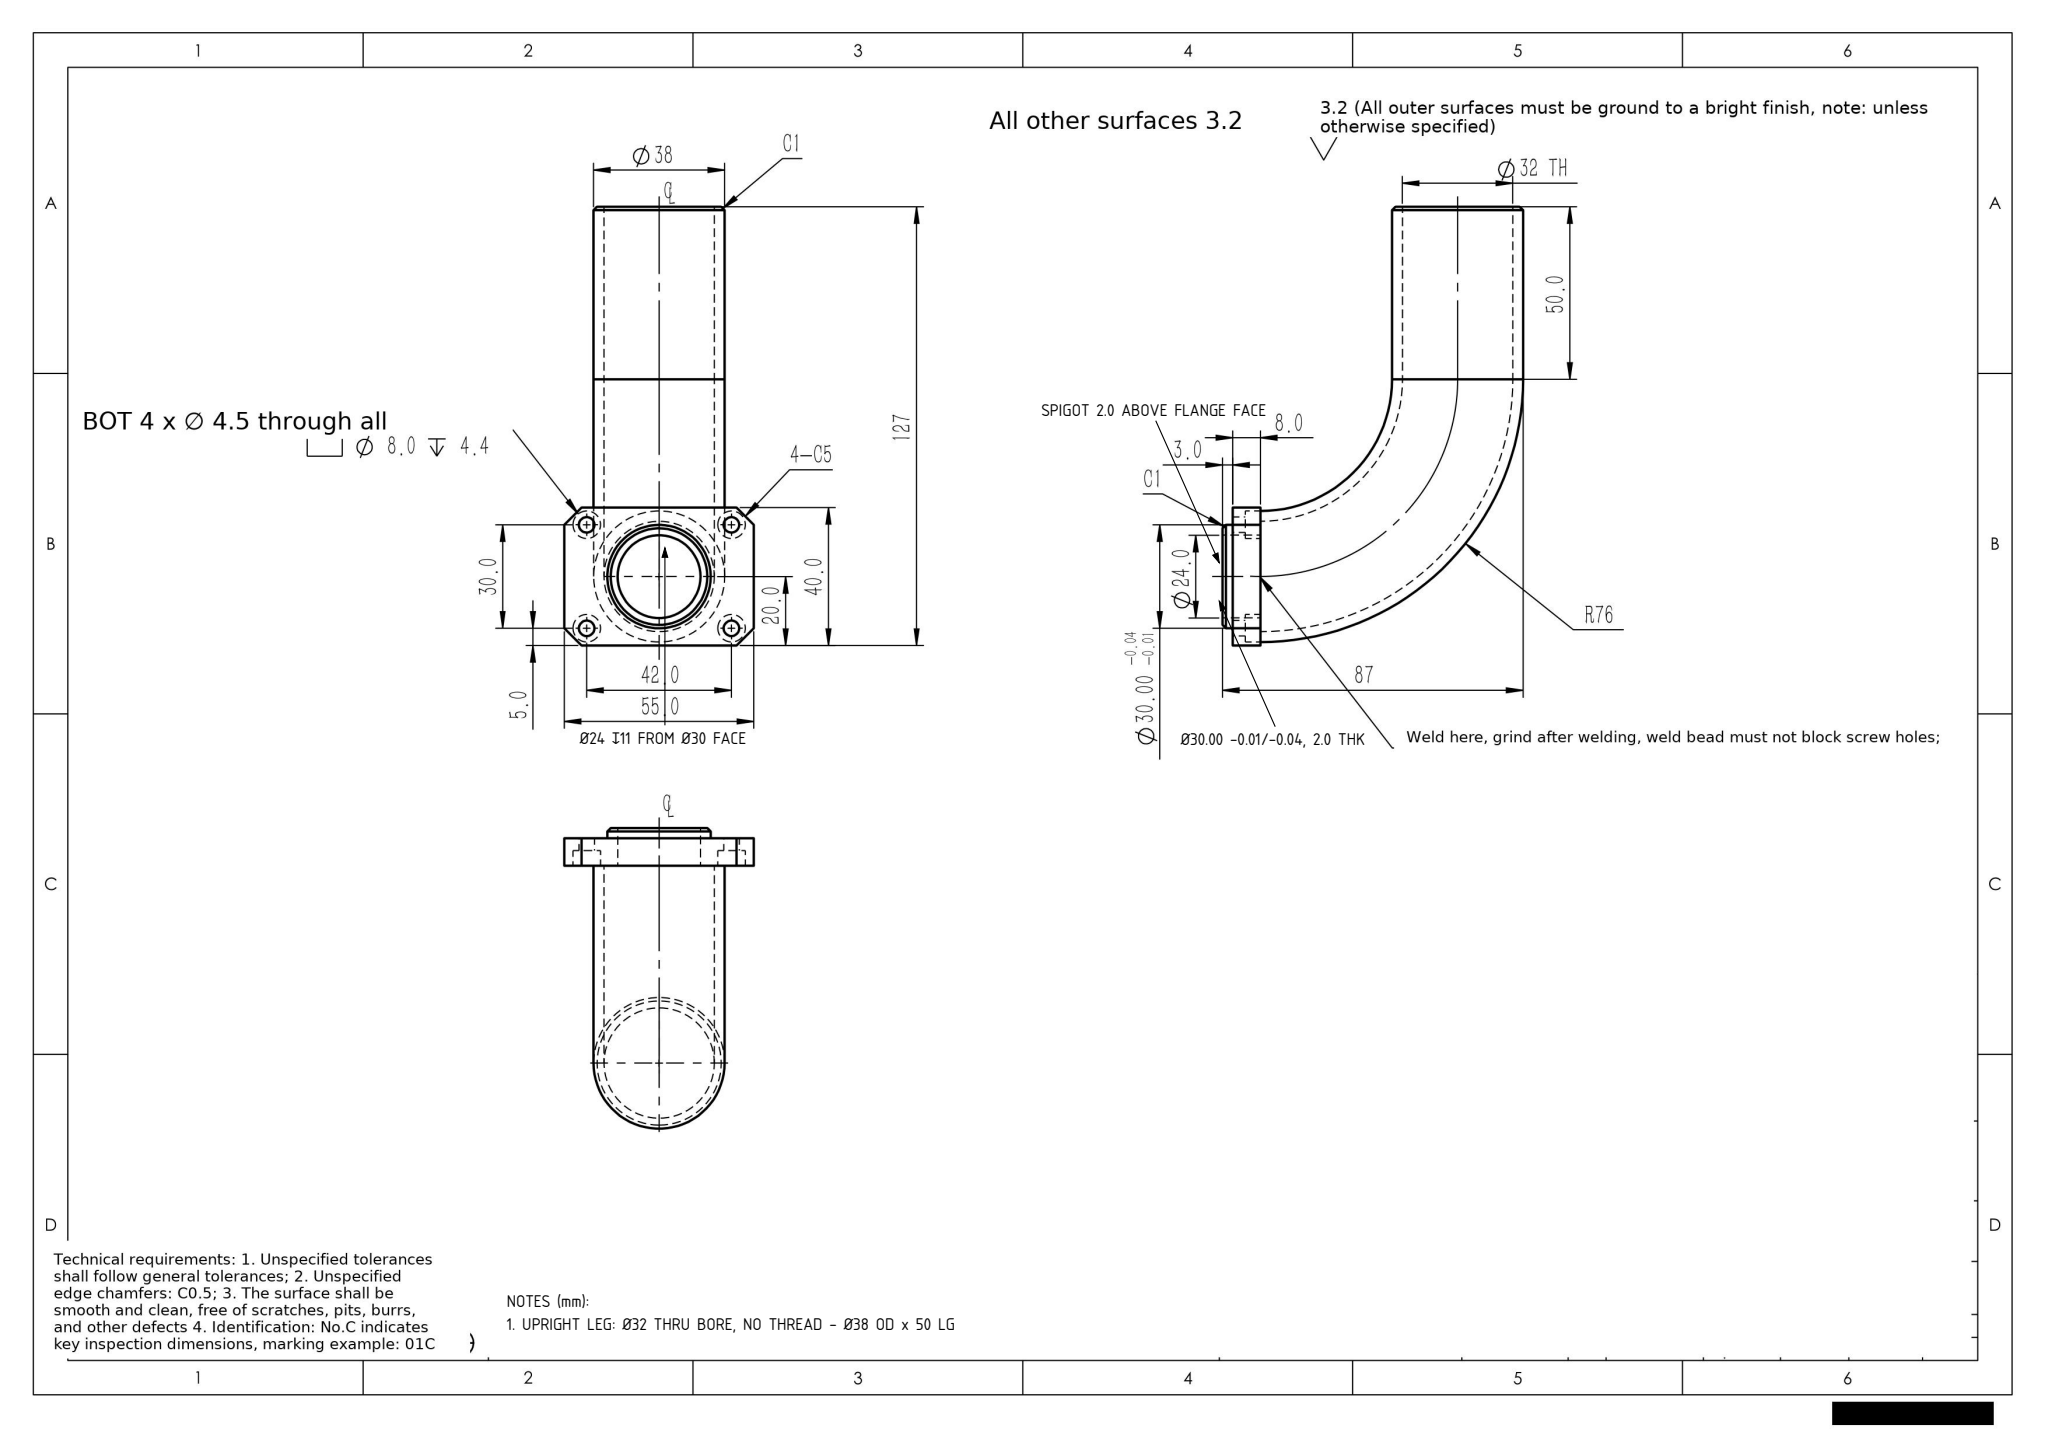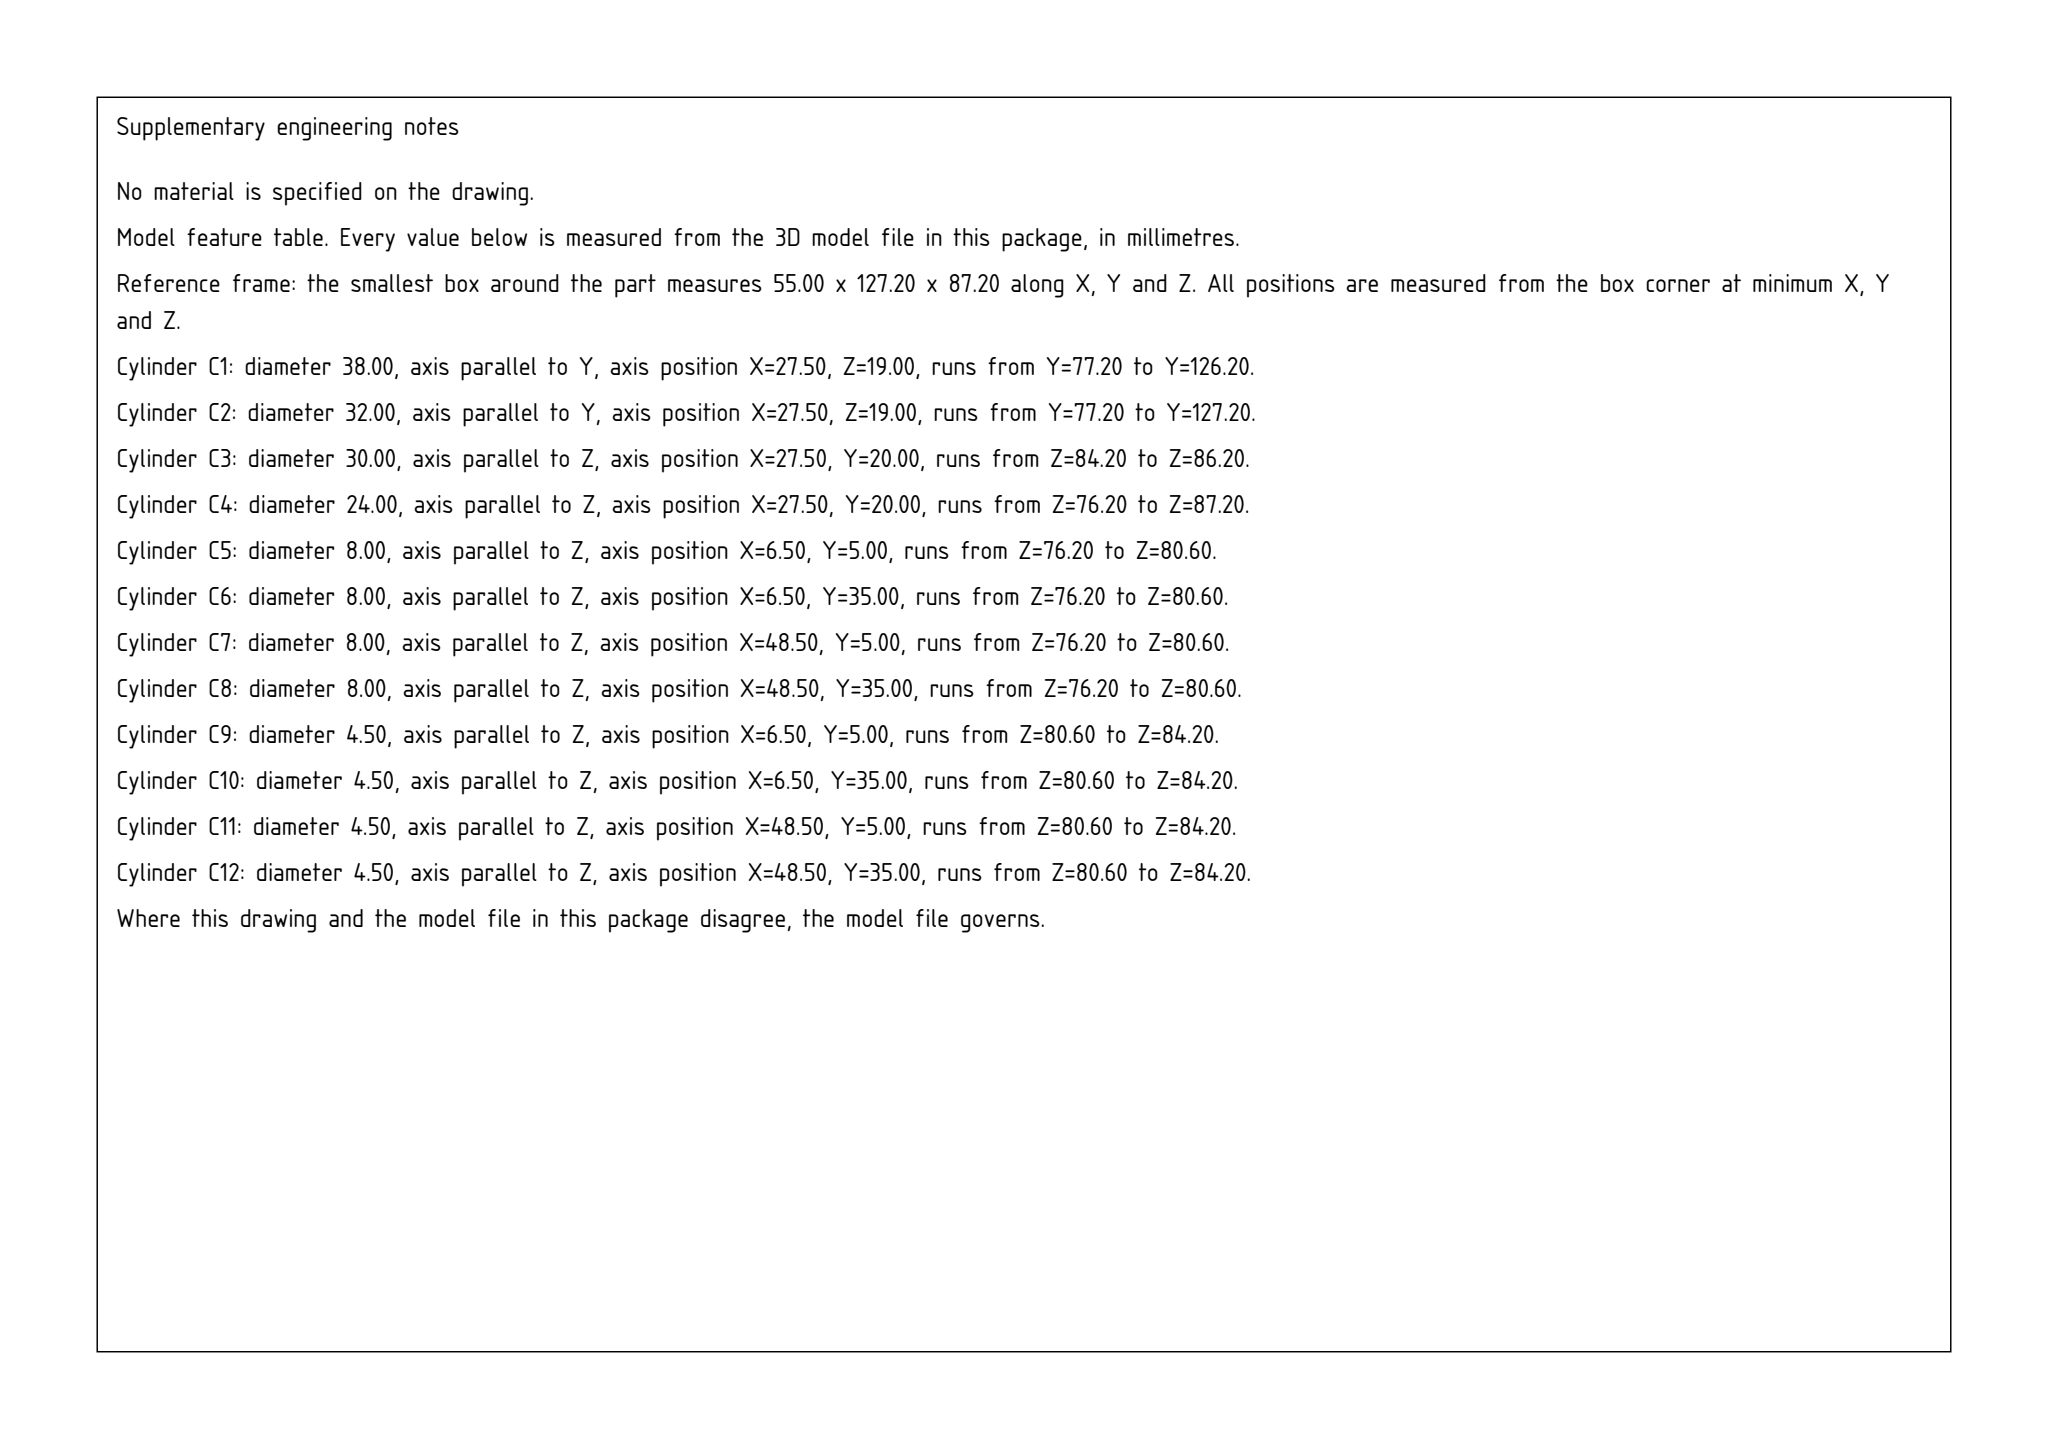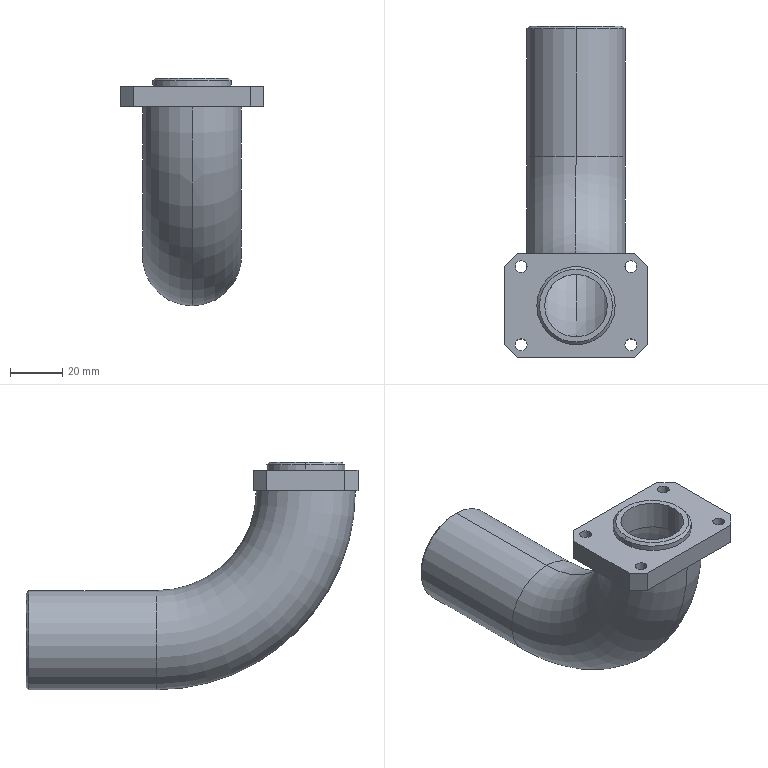Part | SolidWorks | mm | 1 solid | 49 faces | box 55 x 127.2 x 87.2 mm | volume 59258 mm3 | cylinder 24 | plane 17 | torus 4 | cone 4 | commonest cylinder face diameters 8 x8 4.5 x8 32 x2 38 x2 30 x2 24 x2
Drawing notes:
SPIGOT Ø30.00 -0.01/-0.04, 2.0 HIGH ABOVE FLANGE TOP FACE | from the solid: boss/shaft dia 30.0, axis z at (27.5,25.3), z from 90.5 to 92.5 (2.0 above flange top face z=90.5)
UPRIGHT LEG: Ø32 THRU BORE, NO THREAD - Ø38 OD x 50 LG | from the solid: hole/bore Ø32 axis y from 82.5 to 132.5 (50 lg), no thread feature; boss/shaft Ø38 axis y 82.5-131.5
Ø30 SPIGOT: Ø30.00 -0.01/-0.04 (Ø29.99/Ø29.96), 2.0 THK | from the solid: boss/shaft dia 30.0 axis z at (27.5,25.3) from 90.5 to 92.5 = 2.0 high above flange face z=90.5
Ø24 BORE 11 DP FROM Ø30 END FACE, BREAKS INTO Ø32 BORE | from the solid: hole/bore Ø24 axis z from 82.5 to 93.5 (11 long); Ø30 boss ends 92.5 + C1 to 93.5; Ø32 bore axis y at z=25.3 starts y=82.5, step plane z=82.5
build123d program:
from build123d import *

# Parameters (mm, degrees)
SKETCH1_W                                       = 55
SKETCH1_H                                       = 40
SKETCH1_R                                       = 12
BOSS_EXTRUDE1_DEPTH                             = 8
SKETCH3_R                                       = 15
SKETCH3_R_2                                     = 12
BOSS_EXTRUDE2_DEPTH                             = 3
M4_HEX_SOCKET_HEAD_CAP_SCREW_CBORE1_D           = 4.5
M4_HEX_SOCKET_HEAD_CAP_SCREW_CBORE1_CBORE_D     = 8
M4_HEX_SOCKET_HEAD_CAP_SCREW_CBORE1_CBORE_DEPTH = 4.4
SKETCH7_R                                       = 19
SKETCH7_R_2                                     = 16
CHAMFER2_SIZE                                   = 1
CHAMFER1_SIZE                                   = 5
CHAMFER3_SIZE                                   = 1


with BuildPart() as part:
    # Sketch1 → Boss-Extrude1 (new body)
    with BuildSketch(Plane.XY):
        Rectangle(SKETCH1_W, SKETCH1_H)
        Circle(SKETCH1_R, mode=Mode.SUBTRACT)
    extrude(amount=BOSS_EXTRUDE1_DEPTH)

    # Sketch3 → Boss-Extrude2 (add)
    with BuildSketch(Plane.XY.offset(8)):
        Circle(SKETCH3_R)
        Circle(SKETCH3_R_2, mode=Mode.SUBTRACT)
    extrude(amount=BOSS_EXTRUDE2_DEPTH)

    # M4 Hex Socket Head Cap Screw CBORE1 (through all)
    with Locations(Plane(origin=(0, 0, 0), x_dir=(-1, 0, 0), z_dir=(0, 0, -1))):
        with Locations((21, 15), (21, -15), (-21, 15), (-21, -15)):
            CounterBoreHole(M4_HEX_SOCKET_HEAD_CAP_SCREW_CBORE1_D / 2, M4_HEX_SOCKET_HEAD_CAP_SCREW_CBORE1_CBORE_D / 2, M4_HEX_SOCKET_HEAD_CAP_SCREW_CBORE1_CBORE_DEPTH)

    # Sweep1: sweep along a path in Sketch6
    with BuildLine(Plane(origin=(0, 0, 0), x_dir=(0, 0, -1), z_dir=(1, 0, 0))) as sweep1_path:
        Line((57.2, 107.2), (57.2, 57.2))
        ThreePointArc((57.2, 57.2), (40.447, 16.753), (0, 0))
    # Sketch7 → Sweep1 (sweep)
    with BuildSketch(Plane.XY):
        Circle(SKETCH7_R)
        Circle(SKETCH7_R_2, mode=Mode.SUBTRACT)
    sweep(path=sweep1_path.line)

    # Chamfer2
    chamfer2_edges = [part.edges().sort_by_distance(p)[0] for p in [
        (-19, 107.2, -57.2),
    ]]
    chamfer(chamfer2_edges, length=CHAMFER2_SIZE)

    # Chamfer1
    chamfer1_edges = [part.edges().sort_by_distance(p)[0] for p in [
        (27.5, -20, 4),
        (-27.5, -20, 4),
        (-27.5, 20, 4),
        (27.5, 20, 4),
    ]]
    chamfer(chamfer1_edges, length=CHAMFER1_SIZE)

    # Chamfer3
    chamfer3_edges = [part.edges().sort_by_distance(p)[0] for p in [
        (-15, 0, 11),
    ]]
    chamfer(chamfer3_edges, length=CHAMFER3_SIZE)


solid = part.part